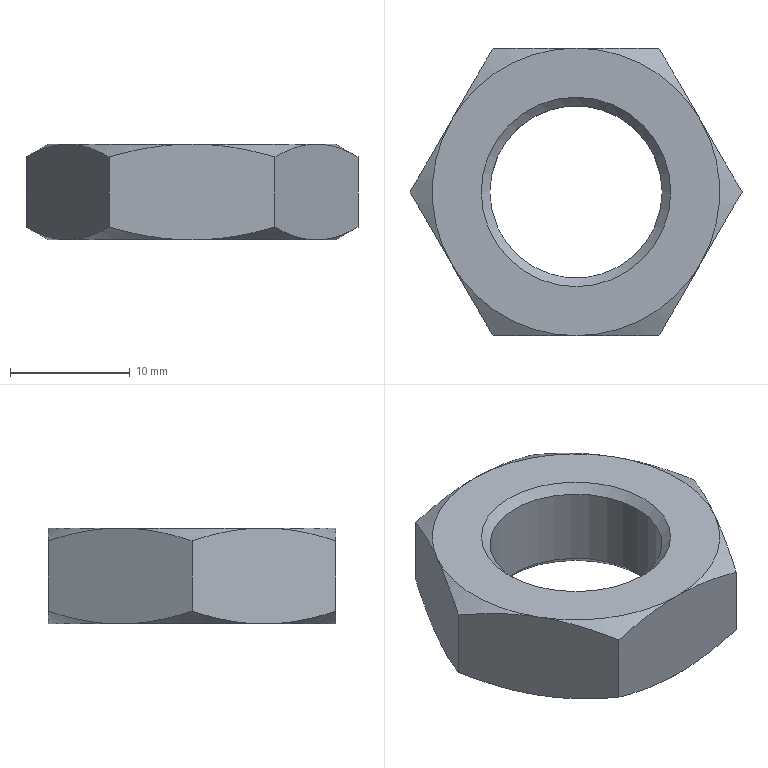Component | NX | GB-T6172_1-2000_M16X2 | 1 solid | 23 faces | volume 2637 mm3 | cone 14 | plane 8 | cylinder 1 | commonest cylinder face diameters 14.376 x1